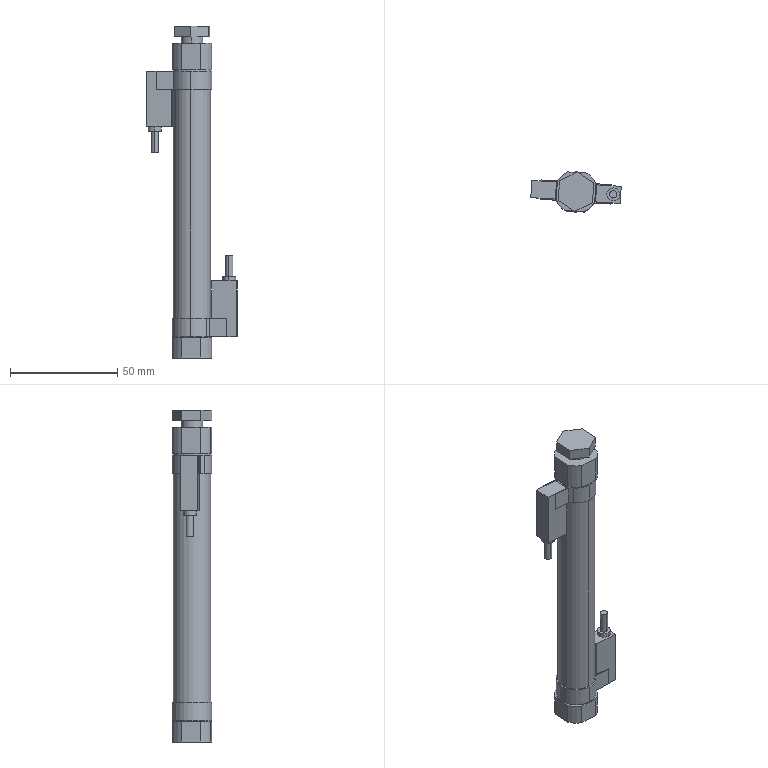Component | SolidWorks | Cylinder-1 | 1 solid | 92 faces | volume 41606 mm3 | plane 58 | cylinder 34 | commonest cylinder face diameters 18.6 x8 20 x8 17.4 x6 6 x4 3.4 x4 10 x2 5.4 x2 | material Plain Carbon Steel